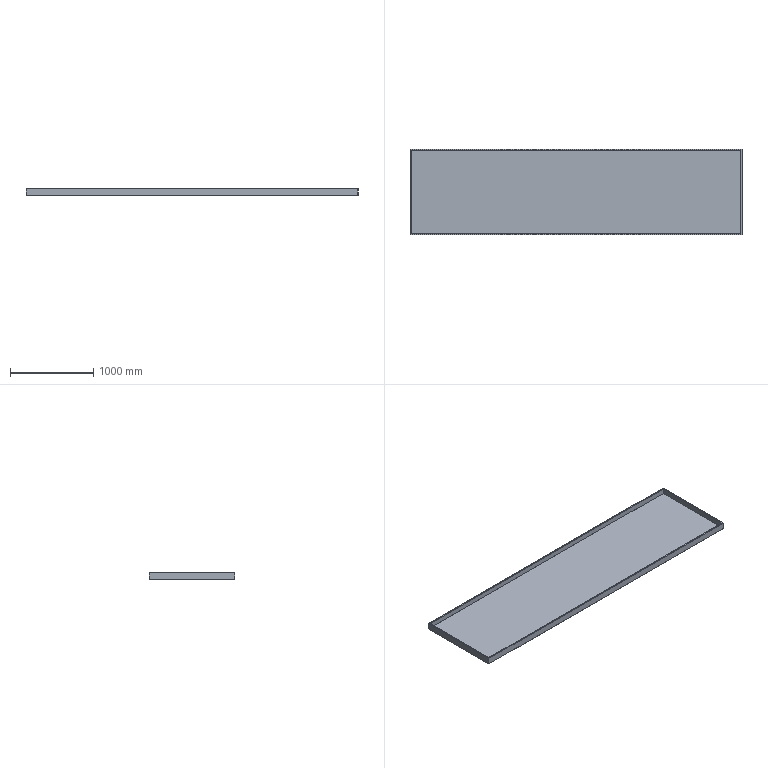Component | NX | DB8_10 | 1 solid | 16 faces | volume 7548027 mm3 | plane 16